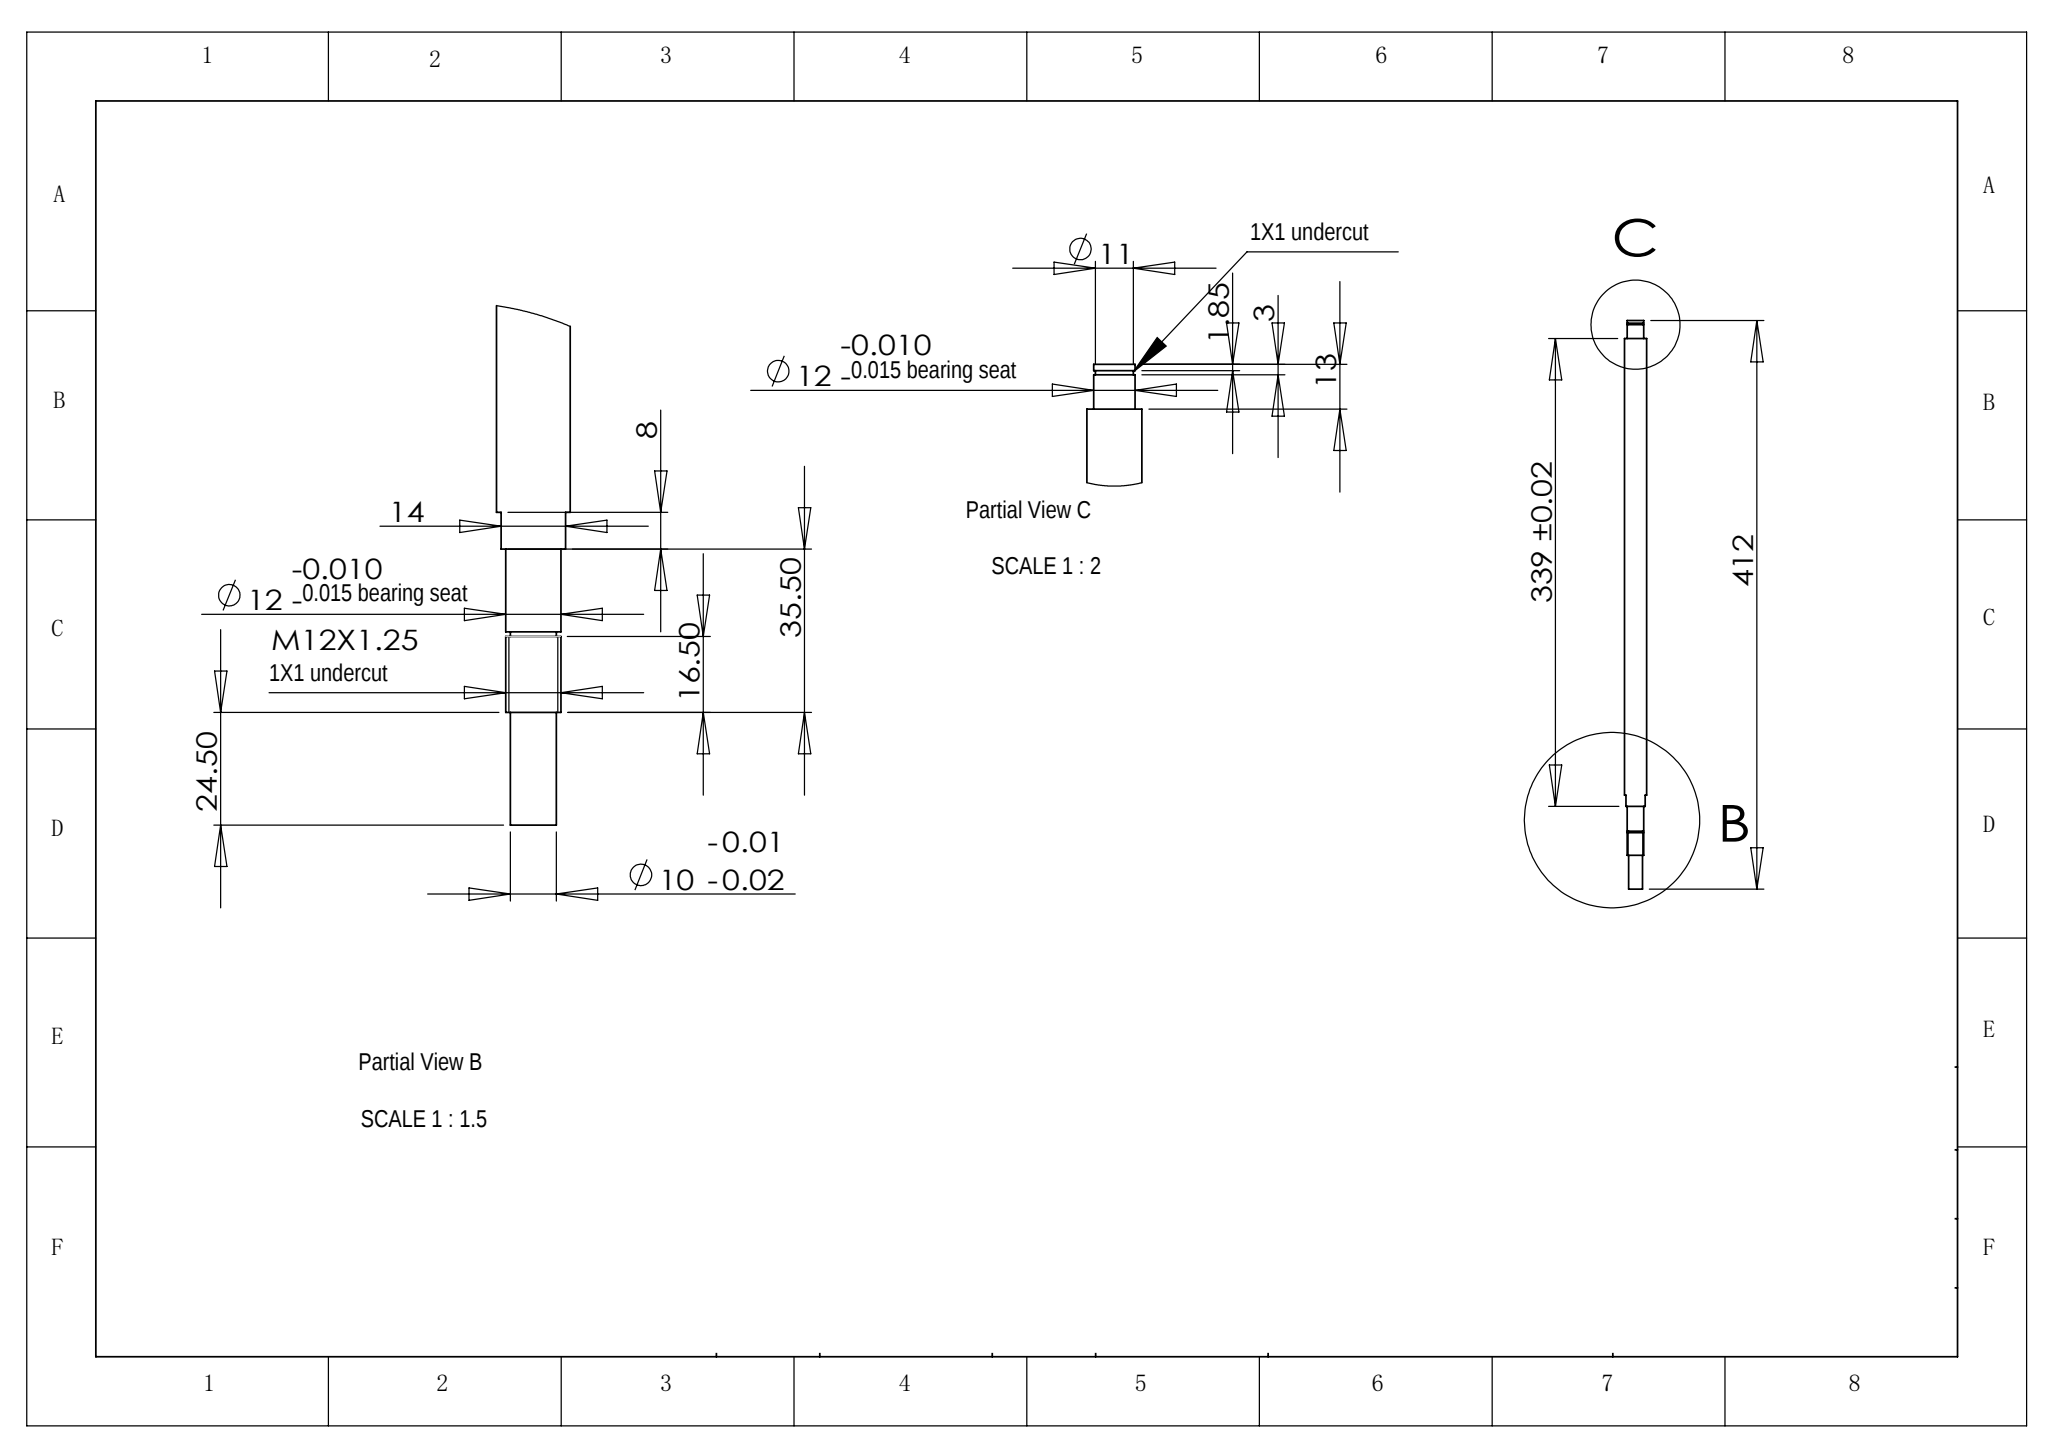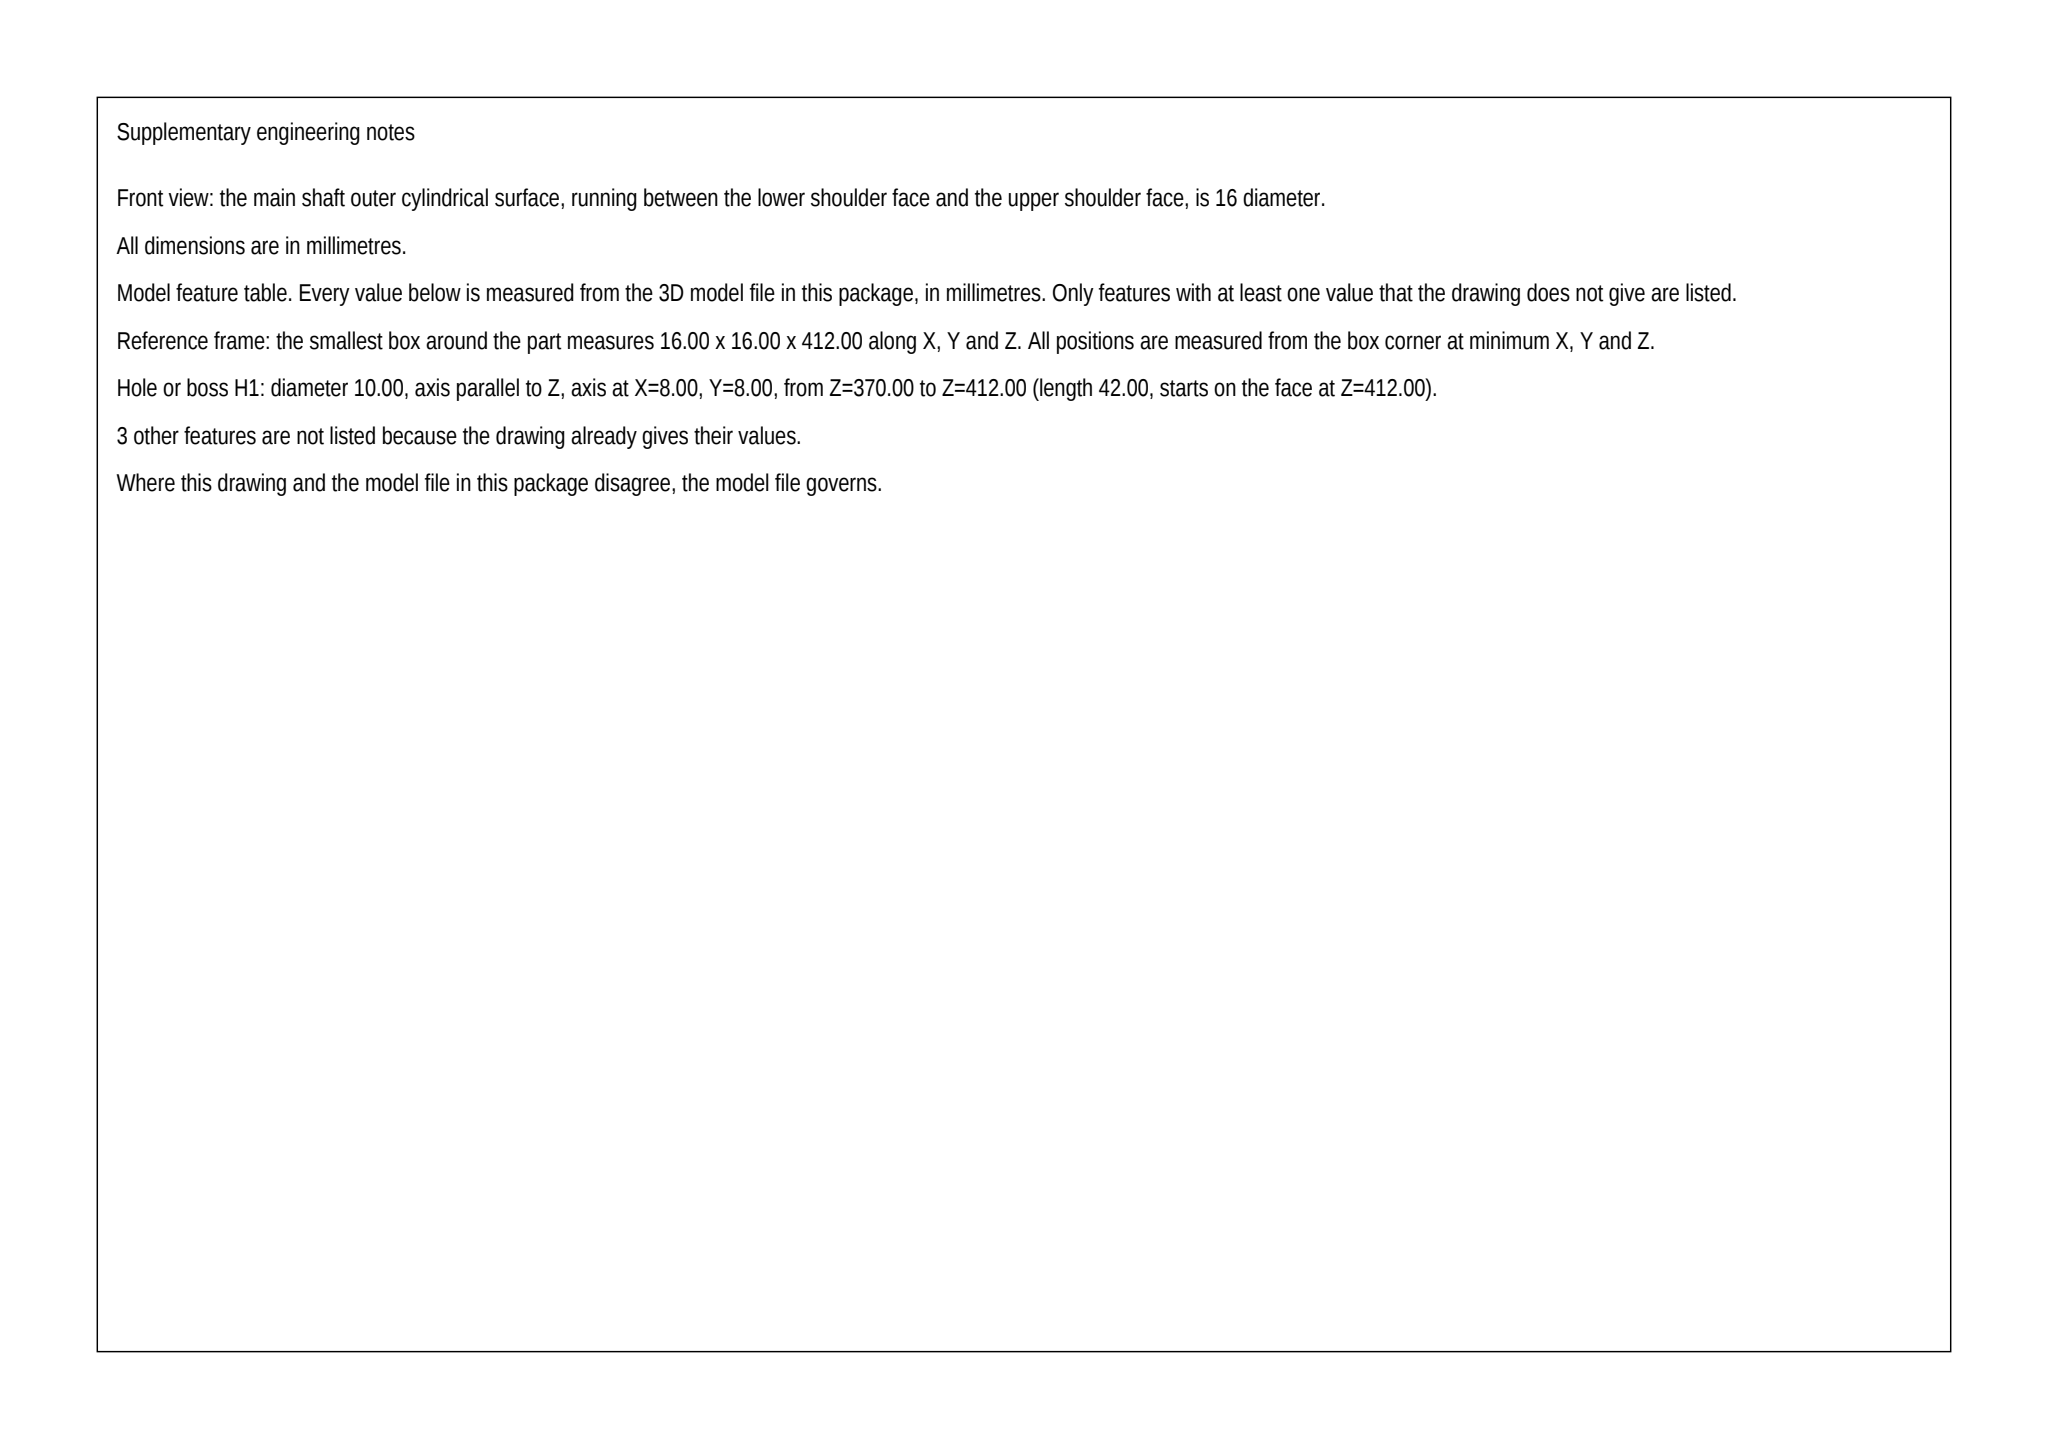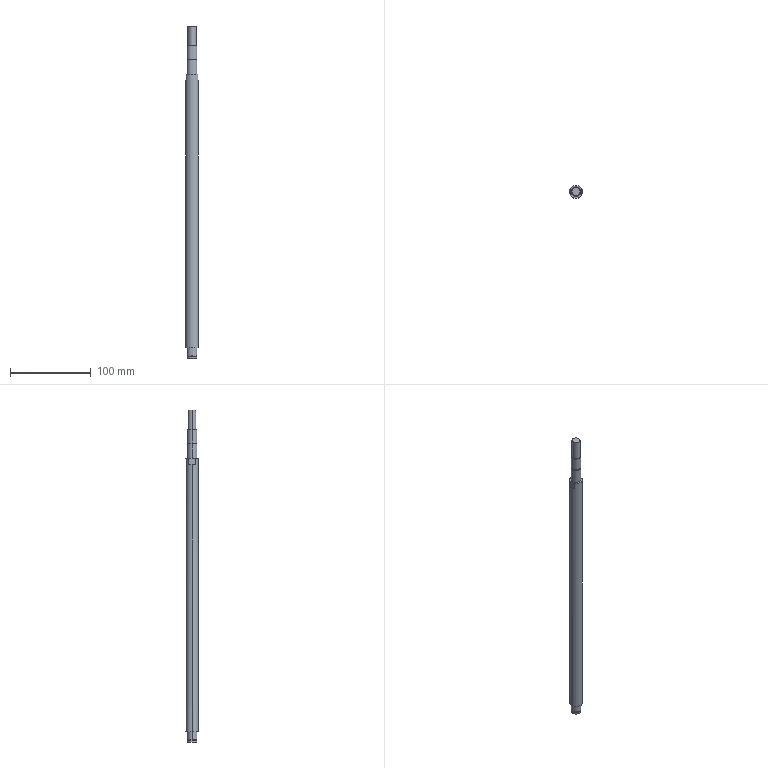Part | SolidWorks | mm | 1 solid | 29 faces | box 16 x 16 x 412 mm | volume 75430 mm3 | cylinder 16 | plane 13 | commonest cylinder face diameters 12 x8 10 x4 11 x2 16 x2
build123d program:
from build123d import *

# Parameters (mm, degrees)
SKETCH1_R               = 8
EXTRUDE1_DEPTH          = 339
SKETCH2_R               = 6
EXTRUDE2_DEPTH          = 13
EXTRUDE3_START          = 35.5
SKETCH3_R               = 6
EXTRUDE3_DEPTH          = 35.5
SKETCH4_R               = 5
EXTRUDE4_DEPTH          = 24.5
CUT_EXTRUDE1_DEPTH      = 10
CUT_EXTRUDE1_DEPTH_BACK = 10
SKETCH6_W               = 13.65
SKETCH6_H               = 12.758
SKETCH6_W_2             = 8.043
SKETCH6_H_2             = 10.569
SKETCH7_W               = 0.5
SKETCH7_H               = 1.15
SKETCH8_W               = 5.586
SKETCH8_H               = 1


with BuildPart() as part:
    # Sketch1 → Extrude1 (new body)
    with BuildSketch(Plane.XY):
        Circle(SKETCH1_R)
    extrude(amount=EXTRUDE1_DEPTH)

    # Sketch2 → Extrude2 (add)
    with BuildSketch(Plane.XY):
        Circle(SKETCH2_R)
    extrude(amount=-EXTRUDE2_DEPTH)

    # Sketch3 → Extrude3 (add)
    with BuildSketch(Plane.XY.offset(339).offset(EXTRUDE3_START)):
        Circle(SKETCH3_R)
    extrude(amount=-EXTRUDE3_DEPTH)

    # Sketch4 → Extrude4 (add)
    with BuildSketch(Plane.XY.offset(374.5)):
        Circle(SKETCH4_R)
    extrude(amount=EXTRUDE4_DEPTH)

    # Sketch6 → Cut-Extrude1 (cut, two sides: drawn at the far end of the back side and taken through both)
    with BuildSketch(Plane(origin=(0, 0, 0), x_dir=(1, 0, 0), z_dir=(0, 1, 0)).offset(-CUT_EXTRUDE1_DEPTH_BACK)):
        with Locations((-13.825, -337.379)):
            Rectangle(SKETCH6_W, SKETCH6_H)
        with Locations((11.021, -336.285)):
            Rectangle(SKETCH6_W_2, SKETCH6_H_2)
    extrude(amount=CUT_EXTRUDE1_DEPTH + CUT_EXTRUDE1_DEPTH_BACK, mode=Mode.SUBTRACT)

    # Sketch7 → Cut-Revolve1 (revolve, cut)
    with BuildSketch(Plane(origin=(0, 0, 0), x_dir=(1, 0, 0), z_dir=(0, 1, 0)), mode=Mode.PRIVATE) as cut_revolve1_sk:
        with Locations((-5.75, 10.575)):
            Rectangle(SKETCH7_W, SKETCH7_H)
    revolve(cut_revolve1_sk.sketch.rotate(Axis((0, 0, -13), (0, 0, 1)), 28.955), axis=Axis((0, 0, -13), (0, 0, 1)), mode=Mode.SUBTRACT)

    # Sketch8 → Cut-Revolve2 (revolve, cut)
    with BuildSketch(Plane(origin=(0, 0, 0), x_dir=(1, 0, 0), z_dir=(0, 1, 0)), mode=Mode.PRIVATE) as cut_revolve2_sk:
        with Locations((7.793, -357.5)):
            Rectangle(SKETCH8_W, SKETCH8_H)
    revolve(cut_revolve2_sk.sketch.rotate(Axis((0, 0, -13), (0, 0, 1)), 180), axis=Axis((0, 0, -13), (0, 0, 1)), mode=Mode.SUBTRACT)


solid = part.part
STEP:
#1=CARTESIAN_POINT('',(6.,0.,374.5));
#2=VERTEX_POINT('',#1);
#3=CARTESIAN_POINT('',(-6.,0.,374.5));
#4=VERTEX_POINT('',#3);
#5=CARTESIAN_POINT('',(0.,0.,374.5));
#6=DIRECTION('',(0.,0.,1.));
#7=DIRECTION('',(1.,0.,0.));
#8=AXIS2_PLACEMENT_3D('',#5,#6,#7);
#9=CIRCLE('',#8,6.);
#10=EDGE_CURVE('',#2,#4,#9,.T.);
#11=ORIENTED_EDGE('',*,*,#10,.F.);
#12=CARTESIAN_POINT('',(6.,0.,358.));
#13=VERTEX_POINT('',#12);
#14=CARTESIAN_POINT('',(6.,0.,374.5));
#15=DIRECTION('',(0.,0.,-1.));
#16=VECTOR('',#15,1000.);
#17=LINE('',#14,#16);
#18=EDGE_CURVE('',#2,#13,#17,.T.);
#19=ORIENTED_EDGE('',*,*,#18,.T.);
#20=CARTESIAN_POINT('',(-6.,0.,358.));
#21=VERTEX_POINT('',#20);
#22=CARTESIAN_POINT('',(0.,0.,358.));
#23=DIRECTION('',(0.,0.,-1.));
#24=DIRECTION('',(-1.,0.,0.));
#25=AXIS2_PLACEMENT_3D('',#22,#23,#24);
#26=CIRCLE('',#25,6.);
#27=EDGE_CURVE('',#21,#13,#26,.T.);
#28=ORIENTED_EDGE('',*,*,#27,.F.);
#29=CARTESIAN_POINT('',(-6.,0.,374.5));
#30=DIRECTION('',(0.,0.,-1.));
#31=VECTOR('',#30,1000.);
#32=LINE('',#29,#31);
#33=EDGE_CURVE('',#4,#21,#32,.T.);
#34=ORIENTED_EDGE('',*,*,#33,.F.);
#35=EDGE_LOOP('',(#11,#19,#28,#34));
#36=FACE_OUTER_BOUND('',#35,.T.);
#37=CARTESIAN_POINT('',(0.,0.,374.5));
#38=DIRECTION('',(0.,0.,-1.));
#39=DIRECTION('',(-1.,0.,0.));
#40=AXIS2_PLACEMENT_3D('',#37,#38,#39);
#41=CYLINDRICAL_SURFACE('',#40,6.);
#42=ADVANCED_FACE('',(#36),#41,.T.);
#43=CARTESIAN_POINT('',(5.,0.,399.));
#44=VERTEX_POINT('',#43);
#45=CARTESIAN_POINT('',(-5.,0.,399.));
#46=VERTEX_POINT('',#45);
#47=CARTESIAN_POINT('',(0.,0.,399.));
#48=DIRECTION('',(0.,0.,1.));
#49=DIRECTION('',(1.,0.,0.));
#50=AXIS2_PLACEMENT_3D('',#47,#48,#49);
#51=CIRCLE('',#50,5.);
#52=EDGE_CURVE('',#44,#46,#51,.T.);
#53=ORIENTED_EDGE('',*,*,#52,.F.);
#54=CARTESIAN_POINT('',(5.,0.,374.5));
#55=VERTEX_POINT('',#54);
#56=CARTESIAN_POINT('',(5.,0.,399.));
#57=DIRECTION('',(0.,0.,-1.));
#58=VECTOR('',#57,1000.);
#59=LINE('',#56,#58);
#60=EDGE_CURVE('',#44,#55,#59,.T.);
#61=ORIENTED_EDGE('',*,*,#60,.T.);
#62=CARTESIAN_POINT('',(-5.,0.,374.5));
#63=VERTEX_POINT('',#62);
#64=CARTESIAN_POINT('',(0.,0.,374.5));
#65=DIRECTION('',(0.,0.,1.));
#66=DIRECTION('',(1.,0.,0.));
#67=AXIS2_PLACEMENT_3D('',#64,#65,#66);
#68=CIRCLE('',#67,5.);
#69=EDGE_CURVE('',#55,#63,#68,.T.);
#70=ORIENTED_EDGE('',*,*,#69,.T.);
#71=CARTESIAN_POINT('',(-5.,0.,399.));
#72=DIRECTION('',(0.,0.,-1.));
#73=VECTOR('',#72,1000.);
#74=LINE('',#71,#73);
#75=EDGE_CURVE('',#46,#63,#74,.T.);
#76=ORIENTED_EDGE('',*,*,#75,.F.);
#77=EDGE_LOOP('',(#53,#61,#70,#76));
#78=FACE_OUTER_BOUND('',#77,.T.);
#79=CARTESIAN_POINT('',(0.,0.,399.));
#80=DIRECTION('',(0.,0.,-1.));
#81=DIRECTION('',(-1.,0.,0.));
#82=AXIS2_PLACEMENT_3D('',#79,#80,#81);
#83=CYLINDRICAL_SURFACE('',#82,5.);
#84=ADVANCED_FACE('',(#78),#83,.T.);
#85=CARTESIAN_POINT('',(-5.,0.,358.));
#86=VERTEX_POINT('',#85);
#87=CARTESIAN_POINT('',(5.,0.,358.));
#88=VERTEX_POINT('',#87);
#89=CARTESIAN_POINT('',(0.,0.,358.));
#90=DIRECTION('',(0.,0.,-1.));
#91=DIRECTION('',(-1.,0.,0.));
#92=AXIS2_PLACEMENT_3D('',#89,#90,#91);
#93=CIRCLE('',#92,5.);
#94=EDGE_CURVE('',#86,#88,#93,.T.);
#95=ORIENTED_EDGE('',*,*,#94,.T.);
#96=CARTESIAN_POINT('',(5.,0.,357.));
#97=VERTEX_POINT('',#96);
#98=CARTESIAN_POINT('',(5.,0.,-13.));
#99=DIRECTION('',(0.,0.,-1.));
#100=VECTOR('',#99,1000.);
#101=LINE('',#98,#100);
#102=EDGE_CURVE('',#88,#97,#101,.T.);
#103=ORIENTED_EDGE('',*,*,#102,.T.);
#104=CARTESIAN_POINT('',(-5.,0.,357.));
#105=VERTEX_POINT('',#104);
#106=CARTESIAN_POINT('',(0.,0.,357.));
#107=DIRECTION('',(0.,0.,-1.));
#108=DIRECTION('',(-1.,0.,0.));
#109=AXIS2_PLACEMENT_3D('',#106,#107,#108);
#110=CIRCLE('',#109,5.);
#111=EDGE_CURVE('',#105,#97,#110,.T.);
#112=ORIENTED_EDGE('',*,*,#111,.F.);
#113=CARTESIAN_POINT('',(-5.,0.,-13.));
#114=DIRECTION('',(0.,0.,-1.));
#115=VECTOR('',#114,1000.);
#116=LINE('',#113,#115);
#117=EDGE_CURVE('',#86,#105,#116,.T.);
#118=ORIENTED_EDGE('',*,*,#117,.F.);
#119=EDGE_LOOP('',(#95,#103,#112,#118));
#120=FACE_OUTER_BOUND('',#119,.T.);
#121=CARTESIAN_POINT('',(0.,0.,-13.));
#122=DIRECTION('',(0.,0.,-1.));
#123=DIRECTION('',(-1.,0.,0.));
#124=AXIS2_PLACEMENT_3D('',#121,#122,#123);
#125=CYLINDRICAL_SURFACE('',#124,5.);
#126=ADVANCED_FACE('',(#120),#125,.T.);
#127=CARTESIAN_POINT('',(6.,0.,-13.));
#128=VERTEX_POINT('',#127);
#129=CARTESIAN_POINT('',(-6.,0.,-13.));
#130=VERTEX_POINT('',#129);
#131=CARTESIAN_POINT('',(0.,0.,-13.));
#132=DIRECTION('',(0.,0.,1.));
#133=DIRECTION('',(1.,0.,0.));
#134=AXIS2_PLACEMENT_3D('',#131,#132,#133);
#135=CIRCLE('',#134,6.);
#136=EDGE_CURVE('',#128,#130,#135,.T.);
#137=ORIENTED_EDGE('',*,*,#136,.T.);
#138=CARTESIAN_POINT('',(-6.,0.,-11.15));
#139=VERTEX_POINT('',#138);
#140=CARTESIAN_POINT('',(-6.,0.,-13.));
#141=DIRECTION('',(0.,0.,1.));
#142=VECTOR('',#141,1000.);
#143=LINE('',#140,#142);
#144=EDGE_CURVE('',#130,#139,#143,.T.);
#145=ORIENTED_EDGE('',*,*,#144,.T.);
#146=CARTESIAN_POINT('',(6.,0.,-11.15));
#147=VERTEX_POINT('',#146);
#148=CARTESIAN_POINT('',(0.,0.,-11.15));
#149=DIRECTION('',(0.,0.,-1.));
#150=DIRECTION('',(-1.,0.,0.));
#151=AXIS2_PLACEMENT_3D('',#148,#149,#150);
#152=CIRCLE('',#151,6.);
#153=EDGE_CURVE('',#139,#147,#152,.T.);
#154=ORIENTED_EDGE('',*,*,#153,.T.);
#155=CARTESIAN_POINT('',(6.,0.,-13.));
#156=DIRECTION('',(0.,0.,1.));
#157=VECTOR('',#156,1000.);
#158=LINE('',#155,#157);
#159=EDGE_CURVE('',#128,#147,#158,.T.);
#160=ORIENTED_EDGE('',*,*,#159,.F.);
#161=EDGE_LOOP('',(#137,#145,#154,#160));
#162=FACE_OUTER_BOUND('',#161,.T.);
#163=CARTESIAN_POINT('',(0.,0.,-13.));
#164=DIRECTION('',(0.,0.,1.));
#165=DIRECTION('',(1.,0.,0.));
#166=AXIS2_PLACEMENT_3D('',#163,#164,#165);
#167=CYLINDRICAL_SURFACE('',#166,6.);
#168=ADVANCED_FACE('',(#162),#167,.T.);
#169=CARTESIAN_POINT('',(-5.5,0.,-10.));
#170=VERTEX_POINT('',#169);
#171=CARTESIAN_POINT('',(5.5,0.,-10.));
#172=VERTEX_POINT('',#171);
#173=CARTESIAN_POINT('',(0.,0.,-10.));
#174=DIRECTION('',(0.,0.,-1.));
#175=DIRECTION('',(-1.,0.,0.));
#176=AXIS2_PLACEMENT_3D('',#173,#174,#175);
#177=CIRCLE('',#176,5.5);
#178=EDGE_CURVE('',#170,#172,#177,.T.);
#179=ORIENTED_EDGE('',*,*,#178,.T.);
#180=CARTESIAN_POINT('',(5.5,0.,-11.15));
#181=VERTEX_POINT('',#180);
#182=CARTESIAN_POINT('',(5.5,0.,-13.));
#183=DIRECTION('',(0.,0.,-1.));
#184=VECTOR('',#183,1000.);
#185=LINE('',#182,#184);
#186=EDGE_CURVE('',#172,#181,#185,.T.);
#187=ORIENTED_EDGE('',*,*,#186,.T.);
#188=CARTESIAN_POINT('',(-5.5,0.,-11.15));
#189=VERTEX_POINT('',#188);
#190=CARTESIAN_POINT('',(0.,0.,-11.15));
#191=DIRECTION('',(0.,0.,-1.));
#192=DIRECTION('',(-1.,0.,0.));
#193=AXIS2_PLACEMENT_3D('',#190,#191,#192);
#194=CIRCLE('',#193,5.5);
#195=EDGE_CURVE('',#189,#181,#194,.T.);
#196=ORIENTED_EDGE('',*,*,#195,.F.);
#197=CARTESIAN_POINT('',(-5.5,0.,-13.));
#198=DIRECTION('',(0.,0.,-1.));
#199=VECTOR('',#198,1000.);
#200=LINE('',#197,#199);
#201=EDGE_CURVE('',#170,#189,#200,.T.);
#202=ORIENTED_EDGE('',*,*,#201,.F.);
#203=EDGE_LOOP('',(#179,#187,#196,#202));
#204=FACE_OUTER_BOUND('',#203,.T.);
#205=CARTESIAN_POINT('',(0.,0.,-13.));
#206=DIRECTION('',(0.,0.,-1.));
#207=DIRECTION('',(-1.,0.,0.));
#208=AXIS2_PLACEMENT_3D('',#205,#206,#207);
#209=CYLINDRICAL_SURFACE('',#208,5.5);
#210=ADVANCED_FACE('',(#204),#209,.T.);
#211=CARTESIAN_POINT('',(8.,0.,331.));
#212=VERTEX_POINT('',#211);
#213=CARTESIAN_POINT('',(7.,3.873,331.));
#214=VERTEX_POINT('',#213);
#215=CARTESIAN_POINT('',(0.,0.,331.));
#216=DIRECTION('',(0.,0.,1.));
#217=DIRECTION('',(1.,0.,0.));
#218=AXIS2_PLACEMENT_3D('',#215,#216,#217);
#219=CIRCLE('',#218,8.);
#220=EDGE_CURVE('',#212,#214,#219,.T.);
#221=ORIENTED_EDGE('',*,*,#220,.F.);
#222=CARTESIAN_POINT('',(8.,0.,0.));
#223=VERTEX_POINT('',#222);
#224=CARTESIAN_POINT('',(8.,0.,339.));
#225=DIRECTION('',(0.,0.,-1.));
#226=VECTOR('',#225,1000.);
#227=LINE('',#224,#226);
#228=EDGE_CURVE('',#212,#223,#227,.T.);
#229=ORIENTED_EDGE('',*,*,#228,.T.);
#230=CARTESIAN_POINT('',(-8.,0.,0.));
#231=VERTEX_POINT('',#230);
#232=CARTESIAN_POINT('',(0.,0.,0.));
#233=DIRECTION('',(0.,0.,1.));
#234=DIRECTION('',(1.,0.,0.));
#235=AXIS2_PLACEMENT_3D('',#232,#233,#234);
#236=CIRCLE('',#235,8.);
#237=EDGE_CURVE('',#223,#231,#236,.T.);
#238=ORIENTED_EDGE('',*,*,#237,.T.);
#239=CARTESIAN_POINT('',(-8.,0.,331.));
#240=VERTEX_POINT('',#239);
#241=CARTESIAN_POINT('',(-8.,0.,339.));
#242=DIRECTION('',(0.,0.,-1.));
#243=VECTOR('',#242,1000.);
#244=LINE('',#241,#243);
#245=EDGE_CURVE('',#240,#231,#244,.T.);
#246=ORIENTED_EDGE('',*,*,#245,.F.);
#247=CARTESIAN_POINT('',(-7.,3.873,331.));
#248=VERTEX_POINT('',#247);
#249=CARTESIAN_POINT('',(0.,0.,331.));
#250=DIRECTION('',(0.,0.,1.));
#251=DIRECTION('',(1.,0.,0.));
#252=AXIS2_PLACEMENT_3D('',#249,#250,#251);
#253=CIRCLE('',#252,8.);
#254=EDGE_CURVE('',#248,#240,#253,.T.);
#255=ORIENTED_EDGE('',*,*,#254,.F.);
#256=CARTESIAN_POINT('',(-7.,3.873,339.));
#257=VERTEX_POINT('',#256);
#258=CARTESIAN_POINT('',(-7.,3.873,339.));
#259=DIRECTION('',(0.,0.,-1.));
#260=VECTOR('',#259,1000.);
#261=LINE('',#258,#260);
#262=EDGE_CURVE('',#257,#248,#261,.T.);
#263=ORIENTED_EDGE('',*,*,#262,.F.);
#264=CARTESIAN_POINT('',(7.,3.873,339.));
#265=VERTEX_POINT('',#264);
#266=CARTESIAN_POINT('',(0.,0.,339.));
#267=DIRECTION('',(0.,0.,1.));
#268=DIRECTION('',(1.,0.,0.));
#269=AXIS2_PLACEMENT_3D('',#266,#267,#268);
#270=CIRCLE('',#269,8.);
#271=EDGE_CURVE('',#265,#257,#270,.T.);
#272=ORIENTED_EDGE('',*,*,#271,.F.);
#273=CARTESIAN_POINT('',(7.,3.873,339.));
#274=DIRECTION('',(0.,0.,1.));
#275=VECTOR('',#274,1000.);
#276=LINE('',#273,#275);
#277=EDGE_CURVE('',#214,#265,#276,.T.);
#278=ORIENTED_EDGE('',*,*,#277,.F.);
#279=EDGE_LOOP('',(#221,#229,#238,#246,#255,#263,#272,#278));
#280=FACE_OUTER_BOUND('',#279,.T.);
#281=CARTESIAN_POINT('',(0.,0.,339.));
#282=DIRECTION('',(0.,0.,-1.));
#283=DIRECTION('',(-1.,0.,0.));
#284=AXIS2_PLACEMENT_3D('',#281,#282,#283);
#285=CYLINDRICAL_SURFACE('',#284,8.);
#286=ADVANCED_FACE('',(#280),#285,.T.);
#287=CARTESIAN_POINT('',(-6.,0.,-10.));
#288=VERTEX_POINT('',#287);
#289=CARTESIAN_POINT('',(6.,0.,-10.));
#290=VERTEX_POINT('',#289);
#291=CARTESIAN_POINT('',(0.,0.,-10.));
#292=DIRECTION('',(0.,0.,-1.));
#293=DIRECTION('',(-1.,0.,0.));
#294=AXIS2_PLACEMENT_3D('',#291,#292,#293);
#295=CIRCLE('',#294,6.);
#296=EDGE_CURVE('',#288,#290,#295,.T.);
#297=ORIENTED_EDGE('',*,*,#296,.F.);
#298=CARTESIAN_POINT('',(-6.,0.,0.));
#299=VERTEX_POINT('',#298);
#300=CARTESIAN_POINT('',(-6.,0.,-13.));
#301=DIRECTION('',(0.,0.,1.));
#302=VECTOR('',#301,1000.);
#303=LINE('',#300,#302);
#304=EDGE_CURVE('',#288,#299,#303,.T.);
#305=ORIENTED_EDGE('',*,*,#304,.T.);
#306=CARTESIAN_POINT('',(6.,0.,0.));
#307=VERTEX_POINT('',#306);
#308=CARTESIAN_POINT('',(0.,0.,0.));
#309=DIRECTION('',(0.,0.,1.));
#310=DIRECTION('',(1.,0.,0.));
#311=AXIS2_PLACEMENT_3D('',#308,#309,#310);
#312=CIRCLE('',#311,6.);
#313=EDGE_CURVE('',#307,#299,#312,.T.);
#314=ORIENTED_EDGE('',*,*,#313,.F.);
#315=CARTESIAN_POINT('',(6.,0.,-13.));
#316=DIRECTION('',(0.,0.,1.));
#317=VECTOR('',#316,1000.);
#318=LINE('',#315,#317);
#319=EDGE_CURVE('',#290,#307,#318,.T.);
#320=ORIENTED_EDGE('',*,*,#319,.F.);
#321=EDGE_LOOP('',(#297,#305,#314,#320));
#322=FACE_OUTER_BOUND('',#321,.T.);
#323=CARTESIAN_POINT('',(0.,0.,-13.));
#324=DIRECTION('',(0.,0.,1.));
#325=DIRECTION('',(1.,0.,0.));
#326=AXIS2_PLACEMENT_3D('',#323,#324,#325);
#327=CYLINDRICAL_SURFACE('',#326,6.);
#328=ADVANCED_FACE('',(#322),#327,.T.);
#329=CARTESIAN_POINT('',(6.,0.,357.));
#330=VERTEX_POINT('',#329);
#331=CARTESIAN_POINT('',(-6.,0.,357.));
#332=VERTEX_POINT('',#331);
#333=CARTESIAN_POINT('',(0.,0.,357.));
#334=DIRECTION('',(0.,0.,1.));
#335=DIRECTION('',(1.,0.,0.));
#336=AXIS2_PLACEMENT_3D('',#333,#334,#335);
#337=CIRCLE('',#336,6.);
#338=EDGE_CURVE('',#330,#332,#337,.T.);
#339=ORIENTED_EDGE('',*,*,#338,.F.);
#340=CARTESIAN_POINT('',(6.,0.,339.));
#341=VERTEX_POINT('',#340);
#342=CARTESIAN_POINT('',(6.,0.,374.5));
#343=DIRECTION('',(0.,0.,-1.));
#344=VECTOR('',#343,1000.);
#345=LINE('',#342,#344);
#346=EDGE_CURVE('',#330,#341,#345,.T.);
#347=ORIENTED_EDGE('',*,*,#346,.T.);
#348=CARTESIAN_POINT('',(-6.,0.,339.));
#349=VERTEX_POINT('',#348);
#350=CARTESIAN_POINT('',(0.,0.,339.));
#351=DIRECTION('',(0.,0.,1.));
#352=DIRECTION('',(1.,0.,0.));
#353=AXIS2_PLACEMENT_3D('',#350,#351,#352);
#354=CIRCLE('',#353,6.);
#355=EDGE_CURVE('',#341,#349,#354,.T.);
#356=ORIENTED_EDGE('',*,*,#355,.T.);
#357=CARTESIAN_POINT('',(-6.,0.,374.5));
#358=DIRECTION('',(0.,0.,-1.));
#359=VECTOR('',#358,1000.);
#360=LINE('',#357,#359);
#361=EDGE_CURVE('',#332,#349,#360,.T.);
#362=ORIENTED_EDGE('',*,*,#361,.F.);
#363=EDGE_LOOP('',(#339,#347,#356,#362));
#364=FACE_OUTER_BOUND('',#363,.T.);
#365=CARTESIAN_POINT('',(0.,0.,374.5));
#366=DIRECTION('',(0.,0.,-1.));
#367=DIRECTION('',(-1.,0.,0.));
#368=AXIS2_PLACEMENT_3D('',#365,#366,#367);
#369=CYLINDRICAL_SURFACE('',#368,6.);
#370=ADVANCED_FACE('',(#364),#369,.T.);
#371=ORIENTED_EDGE('',*,*,#346,.F.);
#372=CARTESIAN_POINT('',(0.,0.,357.));
#373=DIRECTION('',(0.,0.,1.));
#374=DIRECTION('',(1.,0.,0.));
#375=AXIS2_PLACEMENT_3D('',#372,#373,#374);
#376=CIRCLE('',#375,6.);
#377=EDGE_CURVE('',#332,#330,#376,.T.);
#378=ORIENTED_EDGE('',*,*,#377,.F.);
#379=ORIENTED_EDGE('',*,*,#361,.T.);
#380=CARTESIAN_POINT('',(0.,0.,339.));
#381=DIRECTION('',(0.,0.,1.));
#382=DIRECTION('',(1.,0.,0.));
#383=AXIS2_PLACEMENT_3D('',#380,#381,#382);
#384=CIRCLE('',#383,6.);
#385=EDGE_CURVE('',#349,#341,#384,.T.);
#386=ORIENTED_EDGE('',*,*,#385,.T.);
#387=EDGE_LOOP('',(#371,#378,#379,#386));
#388=FACE_OUTER_BOUND('',#387,.T.);
#389=CARTESIAN_POINT('',(0.,0.,374.5));
#390=DIRECTION('',(0.,0.,-1.));
#391=DIRECTION('',(-1.,0.,0.));
#392=AXIS2_PLACEMENT_3D('',#389,#390,#391);
#393=CYLINDRICAL_SURFACE('',#392,6.);
#394=ADVANCED_FACE('',(#388),#393,.T.);
#395=ORIENTED_EDGE('',*,*,#304,.F.);
#396=CARTESIAN_POINT('',(0.,0.,-10.));
#397=DIRECTION('',(0.,0.,-1.));
#398=DIRECTION('',(-1.,0.,0.));
#399=AXIS2_PLACEMENT_3D('',#396,#397,#398);
#400=CIRCLE('',#399,6.);
#401=EDGE_CURVE('',#290,#288,#400,.T.);
#402=ORIENTED_EDGE('',*,*,#401,.F.);
#403=ORIENTED_EDGE('',*,*,#319,.T.);
#404=CARTESIAN_POINT('',(0.,0.,0.));
#405=DIRECTION('',(0.,0.,1.));
#406=DIRECTION('',(1.,0.,0.));
#407=AXIS2_PLACEMENT_3D('',#404,#405,#406);
#408=CIRCLE('',#407,6.);
#409=EDGE_CURVE('',#299,#307,#408,.T.);
#410=ORIENTED_EDGE('',*,*,#409,.F.);
#411=EDGE_LOOP('',(#395,#402,#403,#410));
#412=FACE_OUTER_BOUND('',#411,.T.);
#413=CARTESIAN_POINT('',(0.,0.,-13.));
#414=DIRECTION('',(0.,0.,1.));
#415=DIRECTION('',(1.,0.,0.));
#416=AXIS2_PLACEMENT_3D('',#413,#414,#415);
#417=CYLINDRICAL_SURFACE('',#416,6.);
#418=ADVANCED_FACE('',(#412),#417,.T.);
#419=ORIENTED_EDGE('',*,*,#385,.F.);
#420=ORIENTED_EDGE('',*,*,#355,.F.);
#421=EDGE_LOOP('',(#419,#420));
#422=FACE_BOUND('',#421,.T.);
#423=CARTESIAN_POINT('',(-7.,-3.873,339.));
#424=VERTEX_POINT('',#423);
#425=CARTESIAN_POINT('',(7.,-3.873,339.));
#426=VERTEX_POINT('',#425);
#427=CARTESIAN_POINT('',(0.,0.,339.));
#428=DIRECTION('',(0.,0.,1.));
#429=DIRECTION('',(1.,0.,0.));
#430=AXIS2_PLACEMENT_3D('',#427,#428,#429);
#431=CIRCLE('',#430,8.);
#432=EDGE_CURVE('',#424,#426,#431,.T.);
#433=ORIENTED_EDGE('',*,*,#432,.T.);
#434=CARTESIAN_POINT('',(7.,0.,339.));
#435=DIRECTION('',(0.,1.,0.));
#436=VECTOR('',#435,1000.);
#437=LINE('',#434,#436);
#438=EDGE_CURVE('',#426,#265,#437,.T.);
#439=ORIENTED_EDGE('',*,*,#438,.T.);
#440=ORIENTED_EDGE('',*,*,#271,.T.);
#441=CARTESIAN_POINT('',(-7.,0.,339.));
#442=DIRECTION('',(0.,-1.,0.));
#443=VECTOR('',#442,1000.);
#444=LINE('',#441,#443);
#445=EDGE_CURVE('',#257,#424,#444,.T.);
#446=ORIENTED_EDGE('',*,*,#445,.T.);
#447=EDGE_LOOP('',(#433,#439,#440,#446));
#448=FACE_OUTER_BOUND('',#447,.T.);
#449=CARTESIAN_POINT('',(0.,0.,339.));
#450=DIRECTION('',(0.,0.,1.));
#451=DIRECTION('',(1.,0.,0.));
#452=AXIS2_PLACEMENT_3D('',#449,#450,#451);
#453=PLANE('',#452);
#454=ADVANCED_FACE('',(#422,#448),#453,.T.);
#455=ORIENTED_EDGE('',*,*,#228,.F.);
#456=CARTESIAN_POINT('',(7.,-3.873,331.));
#457=VERTEX_POINT('',#456);
#458=CARTESIAN_POINT('',(0.,0.,331.));
#459=DIRECTION('',(0.,0.,1.));
#460=DIRECTION('',(1.,0.,0.));
#461=AXIS2_PLACEMENT_3D('',#458,#459,#460);
#462=CIRCLE('',#461,8.);
#463=EDGE_CURVE('',#457,#212,#462,.T.);
#464=ORIENTED_EDGE('',*,*,#463,.F.);
#465=CARTESIAN_POINT('',(7.,-3.873,339.));
#466=DIRECTION('',(0.,0.,-1.));
#467=VECTOR('',#466,1000.);
#468=LINE('',#465,#467);
#469=EDGE_CURVE('',#426,#457,#468,.T.);
#470=ORIENTED_EDGE('',*,*,#469,.F.);
#471=ORIENTED_EDGE('',*,*,#432,.F.);
#472=CARTESIAN_POINT('',(-7.,-3.873,331.));
#473=VERTEX_POINT('',#472);
#474=CARTESIAN_POINT('',(-7.,-3.873,339.));
#475=DIRECTION('',(0.,0.,1.));
#476=VECTOR('',#475,1000.);
#477=LINE('',#474,#476);
#478=EDGE_CURVE('',#473,#424,#477,.T.);
#479=ORIENTED_EDGE('',*,*,#478,.F.);
#480=CARTESIAN_POINT('',(0.,0.,331.));
#481=DIRECTION('',(0.,0.,1.));
#482=DIRECTION('',(1.,0.,0.));
#483=AXIS2_PLACEMENT_3D('',#480,#481,#482);
#484=CIRCLE('',#483,8.);
#485=EDGE_CURVE('',#240,#473,#484,.T.);
#486=ORIENTED_EDGE('',*,*,#485,.F.);
#487=ORIENTED_EDGE('',*,*,#245,.T.);
#488=CARTESIAN_POINT('',(0.,0.,0.));
#489=DIRECTION('',(0.,0.,1.));
#490=DIRECTION('',(1.,0.,0.));
#491=AXIS2_PLACEMENT_3D('',#488,#489,#490);
#492=CIRCLE('',#491,8.);
#493=EDGE_CURVE('',#231,#223,#492,.T.);
#494=ORIENTED_EDGE('',*,*,#493,.T.);
#495=EDGE_LOOP('',(#455,#464,#470,#471,#479,#486,#487,#494));
#496=FACE_OUTER_BOUND('',#495,.T.);
#497=CARTESIAN_POINT('',(0.,0.,339.));
#498=DIRECTION('',(0.,0.,-1.));
#499=DIRECTION('',(-1.,0.,0.));
#500=AXIS2_PLACEMENT_3D('',#497,#498,#499);
#501=CYLINDRICAL_SURFACE('',#500,8.);
#502=ADVANCED_FACE('',(#496),#501,.T.);
#503=ORIENTED_EDGE('',*,*,#313,.T.);
#504=ORIENTED_EDGE('',*,*,#409,.T.);
#505=EDGE_LOOP('',(#503,#504));
#506=FACE_BOUND('',#505,.T.);
#507=ORIENTED_EDGE('',*,*,#493,.F.);
#508=ORIENTED_EDGE('',*,*,#237,.F.);
#509=EDGE_LOOP('',(#507,#508));
#510=FACE_OUTER_BOUND('',#509,.T.);
#511=CARTESIAN_POINT('',(0.,0.,0.));
#512=DIRECTION('',(0.,0.,1.));
#513=DIRECTION('',(1.,0.,0.));
#514=AXIS2_PLACEMENT_3D('',#511,#512,#513);
#515=PLANE('',#514);
#516=ADVANCED_FACE('',(#506,#510),#515,.F.);
#517=ORIENTED_EDGE('',*,*,#262,.T.);
#518=CARTESIAN_POINT('',(-7.,10.,331.));
#519=DIRECTION('',(0.,-1.,0.));
#520=VECTOR('',#519,1000.);
#521=LINE('',#518,#520);
#522=EDGE_CURVE('',#248,#473,#521,.T.);
#523=ORIENTED_EDGE('',*,*,#522,.T.);
#524=ORIENTED_EDGE('',*,*,#478,.T.);
#525=ORIENTED_EDGE('',*,*,#445,.F.);
#526=EDGE_LOOP('',(#517,#523,#524,#525));
#527=FACE_OUTER_BOUND('',#526,.T.);
#528=CARTESIAN_POINT('',(-7.,10.,331.));
#529=DIRECTION('',(-1.,0.,-0.));
#530=DIRECTION('',(-0.,0.,1.));
#531=AXIS2_PLACEMENT_3D('',#528,#529,#530);
#532=PLANE('',#531);
#533=ADVANCED_FACE('',(#527),#532,.T.);
#534=ORIENTED_EDGE('',*,*,#254,.T.);
#535=ORIENTED_EDGE('',*,*,#485,.T.);
#536=ORIENTED_EDGE('',*,*,#522,.F.);
#537=EDGE_LOOP('',(#534,#535,#536));
#538=FACE_OUTER_BOUND('',#537,.T.);
#539=CARTESIAN_POINT('',(-20.65,10.,331.));
#540=DIRECTION('',(0.,0.,1.));
#541=DIRECTION('',(1.,0.,0.));
#542=AXIS2_PLACEMENT_3D('',#539,#540,#541);
#543=PLANE('',#542);
#544=ADVANCED_FACE('',(#538),#543,.T.);
#545=ORIENTED_EDGE('',*,*,#469,.T.);
#546=CARTESIAN_POINT('',(7.,10.,331.));
#547=DIRECTION('',(0.,-1.,0.));
#548=VECTOR('',#547,1000.);
#549=LINE('',#546,#548);
#550=EDGE_CURVE('',#214,#457,#549,.T.);
#551=ORIENTED_EDGE('',*,*,#550,.F.);
#552=ORIENTED_EDGE('',*,*,#277,.T.);
#553=ORIENTED_EDGE('',*,*,#438,.F.);
#554=EDGE_LOOP('',(#545,#551,#552,#553));
#555=FACE_OUTER_BOUND('',#554,.T.);
#556=CARTESIAN_POINT('',(7.,10.,331.));
#557=DIRECTION('',(1.,0.,-0.));
#558=DIRECTION('',(-0.,0.,-1.));
#559=AXIS2_PLACEMENT_3D('',#556,#557,#558);
#560=PLANE('',#559);
#561=ADVANCED_FACE('',(#555),#560,.T.);
#562=ORIENTED_EDGE('',*,*,#463,.T.);
#563=ORIENTED_EDGE('',*,*,#220,.T.);
#564=ORIENTED_EDGE('',*,*,#550,.T.);
#565=EDGE_LOOP('',(#562,#563,#564));
#566=FACE_OUTER_BOUND('',#565,.T.);
#567=CARTESIAN_POINT('',(7.,10.,331.));
#568=DIRECTION('',(0.,0.,1.));
#569=DIRECTION('',(1.,0.,0.));
#570=AXIS2_PLACEMENT_3D('',#567,#568,#569);
#571=PLANE('',#570);
#572=ADVANCED_FACE('',(#566),#571,.T.);
#573=ORIENTED_EDGE('',*,*,#178,.F.);
#574=CARTESIAN_POINT('',(0.,0.,-10.));
#575=DIRECTION('',(0.,0.,-1.));
#576=DIRECTION('',(-1.,0.,0.));
#577=AXIS2_PLACEMENT_3D('',#574,#575,#576);
#578=CIRCLE('',#577,5.5);
#579=EDGE_CURVE('',#172,#170,#578,.T.);
#580=ORIENTED_EDGE('',*,*,#579,.F.);
#581=EDGE_LOOP('',(#573,#580));
#582=FACE_BOUND('',#581,.T.);
#583=ORIENTED_EDGE('',*,*,#401,.T.);
#584=ORIENTED_EDGE('',*,*,#296,.T.);
#585=EDGE_LOOP('',(#583,#584));
#586=FACE_OUTER_BOUND('',#585,.T.);
#587=CARTESIAN_POINT('',(-6.,0.,-10.));
#588=DIRECTION('',(0.,0.,1.));
#589=DIRECTION('',(1.,0.,0.));
#590=AXIS2_PLACEMENT_3D('',#587,#588,#589);
#591=PLANE('',#590);
#592=ADVANCED_FACE('',(#582,#586),#591,.F.);
#593=ORIENTED_EDGE('',*,*,#186,.F.);
#594=ORIENTED_EDGE('',*,*,#579,.T.);
#595=ORIENTED_EDGE('',*,*,#201,.T.);
#596=CARTESIAN_POINT('',(0.,0.,-11.15));
#597=DIRECTION('',(0.,0.,-1.));
#598=DIRECTION('',(-1.,0.,0.));
#599=AXIS2_PLACEMENT_3D('',#596,#597,#598);
#600=CIRCLE('',#599,5.5);
#601=EDGE_CURVE('',#181,#189,#600,.T.);
#602=ORIENTED_EDGE('',*,*,#601,.F.);
#603=EDGE_LOOP('',(#593,#594,#595,#602));
#604=FACE_OUTER_BOUND('',#603,.T.);
#605=CARTESIAN_POINT('',(0.,0.,-13.));
#606=DIRECTION('',(0.,0.,-1.));
#607=DIRECTION('',(-1.,0.,0.));
#608=AXIS2_PLACEMENT_3D('',#605,#606,#607);
#609=CYLINDRICAL_SURFACE('',#608,5.5);
#610=ADVANCED_FACE('',(#604),#609,.T.);
#611=CARTESIAN_POINT('',(0.,0.,-11.15));
#612=DIRECTION('',(0.,0.,-1.));
#613=DIRECTION('',(-1.,0.,0.));
#614=AXIS2_PLACEMENT_3D('',#611,#612,#613);
#615=CIRCLE('',#614,6.);
#616=EDGE_CURVE('',#147,#139,#615,.T.);
#617=ORIENTED_EDGE('',*,*,#616,.F.);
#618=ORIENTED_EDGE('',*,*,#153,.F.);
#619=EDGE_LOOP('',(#617,#618));
#620=FACE_OUTER_BOUND('',#619,.T.);
#621=ORIENTED_EDGE('',*,*,#195,.T.);
#622=ORIENTED_EDGE('',*,*,#601,.T.);
#623=EDGE_LOOP('',(#621,#622));
#624=FACE_BOUND('',#623,.T.);
#625=CARTESIAN_POINT('',(-5.5,0.,-11.15));
#626=DIRECTION('',(0.,0.,-1.));
#627=DIRECTION('',(-1.,0.,0.));
#628=AXIS2_PLACEMENT_3D('',#625,#626,#627);
#629=PLANE('',#628);
#630=ADVANCED_FACE('',(#620,#624),#629,.F.);
#631=ORIENTED_EDGE('',*,*,#136,.F.);
#632=CARTESIAN_POINT('',(0.,0.,-13.));
#633=DIRECTION('',(0.,0.,1.));
#634=DIRECTION('',(1.,0.,0.));
#635=AXIS2_PLACEMENT_3D('',#632,#633,#634);
#636=CIRCLE('',#635,6.);
#637=EDGE_CURVE('',#130,#128,#636,.T.);
#638=ORIENTED_EDGE('',*,*,#637,.F.);
#639=EDGE_LOOP('',(#631,#638));
#640=FACE_OUTER_BOUND('',#639,.T.);
#641=CARTESIAN_POINT('',(0.,0.,-13.));
#642=DIRECTION('',(0.,0.,1.));
#643=DIRECTION('',(1.,0.,0.));
#644=AXIS2_PLACEMENT_3D('',#641,#642,#643);
#645=PLANE('',#644);
#646=ADVANCED_FACE('',(#640),#645,.F.);
#647=ORIENTED_EDGE('',*,*,#144,.F.);
#648=ORIENTED_EDGE('',*,*,#637,.T.);
#649=ORIENTED_EDGE('',*,*,#159,.T.);
#650=ORIENTED_EDGE('',*,*,#616,.T.);
#651=EDGE_LOOP('',(#647,#648,#649,#650));
#652=FACE_OUTER_BOUND('',#651,.T.);
#653=CARTESIAN_POINT('',(0.,0.,-13.));
#654=DIRECTION('',(0.,0.,1.));
#655=DIRECTION('',(1.,0.,0.));
#656=AXIS2_PLACEMENT_3D('',#653,#654,#655);
#657=CYLINDRICAL_SURFACE('',#656,6.);
#658=ADVANCED_FACE('',(#652),#657,.T.);
#659=ORIENTED_EDGE('',*,*,#94,.F.);
#660=CARTESIAN_POINT('',(0.,0.,358.));
#661=DIRECTION('',(0.,0.,-1.));
#662=DIRECTION('',(-1.,0.,0.));
#663=AXIS2_PLACEMENT_3D('',#660,#661,#662);
#664=CIRCLE('',#663,5.);
#665=EDGE_CURVE('',#88,#86,#664,.T.);
#666=ORIENTED_EDGE('',*,*,#665,.F.);
#667=EDGE_LOOP('',(#659,#666));
#668=FACE_BOUND('',#667,.T.);
#669=ORIENTED_EDGE('',*,*,#27,.T.);
#670=CARTESIAN_POINT('',(0.,0.,358.));
#671=DIRECTION('',(0.,0.,-1.));
#672=DIRECTION('',(-1.,0.,0.));
#673=AXIS2_PLACEMENT_3D('',#670,#671,#672);
#674=CIRCLE('',#673,6.);
#675=EDGE_CURVE('',#13,#21,#674,.T.);
#676=ORIENTED_EDGE('',*,*,#675,.T.);
#677=EDGE_LOOP('',(#669,#676));
#678=FACE_OUTER_BOUND('',#677,.T.);
#679=CARTESIAN_POINT('',(5.,0.,358.));
#680=DIRECTION('',(0.,0.,-1.));
#681=DIRECTION('',(-1.,0.,0.));
#682=AXIS2_PLACEMENT_3D('',#679,#680,#681);
#683=PLANE('',#682);
#684=ADVANCED_FACE('',(#668,#678),#683,.T.);
#685=ORIENTED_EDGE('',*,*,#111,.T.);
#686=CARTESIAN_POINT('',(0.,0.,357.));
#687=DIRECTION('',(0.,0.,-1.));
#688=DIRECTION('',(-1.,0.,0.));
#689=AXIS2_PLACEMENT_3D('',#686,#687,#688);
#690=CIRCLE('',#689,5.);
#691=EDGE_CURVE('',#97,#105,#690,.T.);
#692=ORIENTED_EDGE('',*,*,#691,.T.);
#693=EDGE_LOOP('',(#685,#692));
#694=FACE_BOUND('',#693,.T.);
#695=ORIENTED_EDGE('',*,*,#377,.T.);
#696=ORIENTED_EDGE('',*,*,#338,.T.);
#697=EDGE_LOOP('',(#695,#696));
#698=FACE_OUTER_BOUND('',#697,.T.);
#699=CARTESIAN_POINT('',(5.,0.,357.));
#700=DIRECTION('',(0.,0.,1.));
#701=DIRECTION('',(1.,0.,0.));
#702=AXIS2_PLACEMENT_3D('',#699,#700,#701);
#703=PLANE('',#702);
#704=ADVANCED_FACE('',(#694,#698),#703,.T.);
#705=ORIENTED_EDGE('',*,*,#102,.F.);
#706=ORIENTED_EDGE('',*,*,#665,.T.);
#707=ORIENTED_EDGE('',*,*,#117,.T.);
#708=ORIENTED_EDGE('',*,*,#691,.F.);
#709=EDGE_LOOP('',(#705,#706,#707,#708));
#710=FACE_OUTER_BOUND('',#709,.T.);
#711=CARTESIAN_POINT('',(0.,0.,-13.));
#712=DIRECTION('',(0.,0.,-1.));
#713=DIRECTION('',(-1.,0.,0.));
#714=AXIS2_PLACEMENT_3D('',#711,#712,#713);
#715=CYLINDRICAL_SURFACE('',#714,5.);
#716=ADVANCED_FACE('',(#710),#715,.T.);
#717=CARTESIAN_POINT('',(0.,0.,399.));
#718=DIRECTION('',(0.,0.,1.));
#719=DIRECTION('',(1.,0.,0.));
#720=AXIS2_PLACEMENT_3D('',#717,#718,#719);
#721=CIRCLE('',#720,5.);
#722=EDGE_CURVE('',#46,#44,#721,.T.);
#723=ORIENTED_EDGE('',*,*,#722,.T.);
#724=ORIENTED_EDGE('',*,*,#52,.T.);
#725=EDGE_LOOP('',(#723,#724));
#726=FACE_OUTER_BOUND('',#725,.T.);
#727=CARTESIAN_POINT('',(0.,0.,399.));
#728=DIRECTION('',(0.,0.,1.));
#729=DIRECTION('',(1.,0.,0.));
#730=AXIS2_PLACEMENT_3D('',#727,#728,#729);
#731=PLANE('',#730);
#732=ADVANCED_FACE('',(#726),#731,.T.);
#733=ORIENTED_EDGE('',*,*,#60,.F.);
#734=ORIENTED_EDGE('',*,*,#722,.F.);
#735=ORIENTED_EDGE('',*,*,#75,.T.);
#736=CARTESIAN_POINT('',(0.,0.,374.5));
#737=DIRECTION('',(0.,0.,1.));
#738=DIRECTION('',(1.,0.,0.));
#739=AXIS2_PLACEMENT_3D('',#736,#737,#738);
#740=CIRCLE('',#739,5.);
#741=EDGE_CURVE('',#63,#55,#740,.T.);
#742=ORIENTED_EDGE('',*,*,#741,.T.);
#743=EDGE_LOOP('',(#733,#734,#735,#742));
#744=FACE_OUTER_BOUND('',#743,.T.);
#745=CARTESIAN_POINT('',(0.,0.,399.));
#746=DIRECTION('',(0.,0.,-1.));
#747=DIRECTION('',(-1.,0.,0.));
#748=AXIS2_PLACEMENT_3D('',#745,#746,#747);
#749=CYLINDRICAL_SURFACE('',#748,5.);
#750=ADVANCED_FACE('',(#744),#749,.T.);
#751=CARTESIAN_POINT('',(0.,0.,374.5));
#752=DIRECTION('',(0.,0.,1.));
#753=DIRECTION('',(1.,0.,0.));
#754=AXIS2_PLACEMENT_3D('',#751,#752,#753);
#755=CIRCLE('',#754,6.);
#756=EDGE_CURVE('',#4,#2,#755,.T.);
#757=ORIENTED_EDGE('',*,*,#756,.T.);
#758=ORIENTED_EDGE('',*,*,#10,.T.);
#759=EDGE_LOOP('',(#757,#758));
#760=FACE_OUTER_BOUND('',#759,.T.);
#761=ORIENTED_EDGE('',*,*,#741,.F.);
#762=ORIENTED_EDGE('',*,*,#69,.F.);
#763=EDGE_LOOP('',(#761,#762));
#764=FACE_BOUND('',#763,.T.);
#765=CARTESIAN_POINT('',(0.,0.,374.5));
#766=DIRECTION('',(0.,0.,1.));
#767=DIRECTION('',(1.,0.,0.));
#768=AXIS2_PLACEMENT_3D('',#765,#766,#767);
#769=PLANE('',#768);
#770=ADVANCED_FACE('',(#760,#764),#769,.T.);
#771=ORIENTED_EDGE('',*,*,#18,.F.);
#772=ORIENTED_EDGE('',*,*,#756,.F.);
#773=ORIENTED_EDGE('',*,*,#33,.T.);
#774=ORIENTED_EDGE('',*,*,#675,.F.);
#775=EDGE_LOOP('',(#771,#772,#773,#774));
#776=FACE_OUTER_BOUND('',#775,.T.);
#777=CARTESIAN_POINT('',(0.,0.,374.5));
#778=DIRECTION('',(0.,0.,-1.));
#779=DIRECTION('',(-1.,0.,0.));
#780=AXIS2_PLACEMENT_3D('',#777,#778,#779);
#781=CYLINDRICAL_SURFACE('',#780,6.);
#782=ADVANCED_FACE('',(#776),#781,.T.);
#783=CLOSED_SHELL('',(#42,#84,#126,#168,#210,#286,#328,#370,#394,#418,#454,#502,#516,#533,#544,#561,#572,#592,#610,#630,#646,#658,#684,#704,#716,#732,#750,#770,#782));
#784=MANIFOLD_SOLID_BREP('',#783);
#785=CARTESIAN_POINT('',(0.,0.,0.));
#786=DIRECTION('',(0.,0.,1.));
#787=DIRECTION('',(1.,0.,0.));
#788=AXIS2_PLACEMENT_3D('',#785,#786,#787);
#789=(LENGTH_UNIT()NAMED_UNIT(*)SI_UNIT(.MILLI.,.METRE.));
#790=UNCERTAINTY_MEASURE_WITH_UNIT(LENGTH_MEASURE(0.00001),#789,'','');
#791=(NAMED_UNIT(*)PLANE_ANGLE_UNIT()SI_UNIT($,.RADIAN.));
#792=(NAMED_UNIT(*)SI_UNIT($,.STERADIAN.)SOLID_ANGLE_UNIT());
#793=(GEOMETRIC_REPRESENTATION_CONTEXT(3)GLOBAL_UNCERTAINTY_ASSIGNED_CONTEXT((#790))GLOBAL_UNIT_ASSIGNED_CONTEXT((#789,#791,#792))REPRESENTATION_CONTEXT('',''));
#794=ADVANCED_BREP_SHAPE_REPRESENTATION('',(#784,#788),#793);